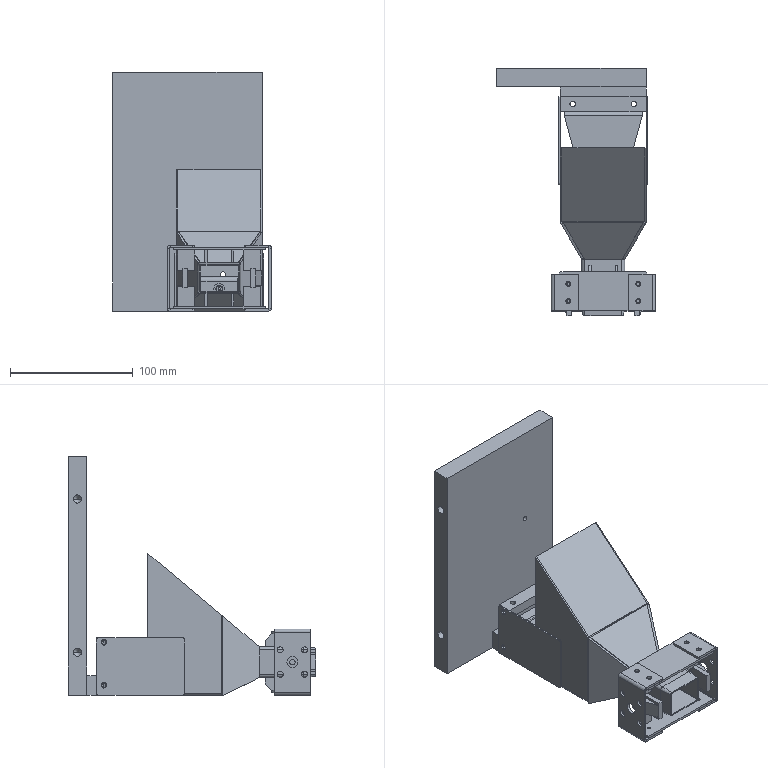Assembly | SolidWorks | mm | 12 component files | 29 solids | 449 faces | box 129.5 x 201.89 x 195.59 mm | volume 479848 mm3 | plane 263 | cylinder 162 | cone 18 | spline 4 | sphere 2 | commonest cylinder face diameters 4.5 x24 5 x24 4 x24 2.5 x16 3.3 x14 2 x14 1 x12 4.2 x8
Bill of materials:
InnerBagFunnel1 | 1 |  | Multi-body fabricated-style assembly: a rectangular hollow tube with rounded corners runs between two parallel flat plates, with small vertical rib plates between the plates. One end of the tube opens into a flared, pyramid-shaped (funnel-like) rectangular transition. The other end narrows slightly.
InnerBagFunnel2 | 1 |  | Bent thin-wall (sheet-like) part: a rectangular open channel or box section with one end cut at an angle, plus a flat tab extending sideways with two holes. A semicircular notch is cut into the edge of the bottom panel.
ClampingBlock | 2 |  | Solid prismatic block with a tapered lower profile, one round through-hole, a rectangular notch cut across the top edge, opposing notches on the sides, and a shallow rectangular recess or step on one face.
InnerBagClampingCylinderFixingPlate | 2 |  | U-shaped (C-channel) thin bracket with rounded bends. The web has one large central hole and four smaller holes in a rectangular pattern. Each of the two parallel flanges has two holes.
InnerBagLiftingAluminumBlockA | 1 |  | Rectangular solid bar with several cross-drilled holes: two holes through the top face near each end, two holes through a side face near each end, and one hole at the end face.
InnerBagLiftingAluminumBlockB | 1 |  | Rectangular solid bar with two through-holes in the top face near each end and one hole in an end face. No holes are visible on the long side face.
InnerBagLiftingCylinderFixingPlate | 1 |  | Flat rectangular plate with two small round holes, both near one long edge.
SiliconeShockAbsorberBlock | 1 |  | Plain rectangular solid bar with no visible holes or other features.
SmallRoundCylinderBracket | 1 |  | Bent thin bracket with a trapezoidal (tapered) top panel and two downturned legs with rounded bends. The legs have unequal lengths, and each has one round hole.
TeaSortingRod | 1 |  | Pin-like revolved part: a short cylindrical head with chamfered ends and a long, slender, coaxial cylindrical shaft ending in a rounded tip.
Mates:
1. coincident | InnerBagLiftingCylinderFixingPlate-1 face at (-22.646, -34.068, 148.933) dir (0, -1, 0) | assembly face at (71.854, 23.397, 163.933) dir (0, 0, -1)
2. concentric | InnerBagLiftingCylinderFixingPlate-1 face at (67.354, -34.068, 258.933) dir (0, -1, 0) r 2.1 | assembly face at (64.354, 133.397, 183.633) dir (0, 0, -1) r 2.6
3. concentric | InnerBagLiftingCylinderFixingPlate-1 face at (67.354, -34.068, 178.933) dir (0, -1, 0) r 2.1 | assembly face at (64.354, 53.397, 183.633) dir (0, 0, -1) r 2.6
4. coincident | assembly face at (33.354, -54.068, 187.933) dir (0, 0, 1) | InnerBagLiftingAluminumBlockB-1 face at (29.354, -54.068, 187.933) dir (0, 0, -1)
5. concentric | assembly face at (89.354, -48.068, 187.554) dir (0, 0, -1) r 1.621 | InnerBagLiftingAluminumBlockB-1 face at (89.354, -48.068, 187.933) dir (0, 0, 1) r 2.25
6. concentric | assembly face at (39.354, -48.068, 187.554) dir (0, 0, -1) r 1.621 | InnerBagLiftingAluminumBlockB-1 face at (39.354, -48.068, 187.933) dir (0, 0, 1) r 2.25
7. coincident | assembly face at (95.354, -54.068, 164.933) dir (0, 0, -1) | InnerBagLiftingAluminumBlockA-1 face at (29.354, -54.068, 164.933) dir (0, 0, 1)
8. concentric | InnerBagLiftingAluminumBlockA-1 face at (89.354, -48.068, 148.933) dir (0, 0, 1) r 2.25 | InnerBagLiftingAluminumBlockB-1 face at (89.354, -48.068, 187.933) dir (0, 0, 1) r 2.25
9. concentric | InnerBagLiftingAluminumBlockA-1 face at (39.354, -48.068, 148.933) dir (0, 0, 1) r 2.25 | InnerBagLiftingAluminumBlockB-1 face at (39.354, -48.068, 187.933) dir (0, 0, 1) r 2.25
10. coincident | InnerBagLiftingAluminumBlockA-1 face at (29.354, -54.068, 164.933) dir (0, -1, 0) | SmallRoundCylinderBracket-1 face at (96.354, -54.068, 176.933) dir (0, 1, 0)
11. concentric | InnerBagLiftingAluminumBlockA-1 face at (44.354, -42.068, 156.933) dir (0, 1, 0) r 1.65 | SmallRoundCylinderBracket-1 face at (44.354, -64.068, 156.933) dir (0, 1, 0) r 2.25
12. concentric | InnerBagLiftingAluminumBlockA-1 face at (84.354, -42.068, 156.933) dir (0, 1, 0) r 1.65 | SmallRoundCylinderBracket-1 face at (84.354, -64.068, 156.933) dir (0, 1, 0) r 2.25
13. coincident | InnerBagLiftingAluminumBlockA-1 face at (99.354, -54.068, 164.933) dir (1, 0, 0) | BAssemblyInnerBagFunnel-1/InnerBagFunnel2-1 face at (99.354, -112.068, 150.933) dir (-1, 0, 0)
14. concentric | InnerBagLiftingAluminumBlockA-1 face at (99.354, -48.068, 156.933) dir (1, 0, 0) r 1.65 | BAssemblyInnerBagFunnel-1/InnerBagFunnel2-1 face at (100.554, -48.068, 156.933) dir (-1, 0, 0) r 2.25
15. concentric | InnerBagLiftingAluminumBlockB-1 face at (99.354, -48.068, 191.933) dir (1, 0, 0) r 1.65 | BAssemblyInnerBagFunnel-1/InnerBagFunnel2-1 face at (100.554, -48.068, 191.933) dir (-1, 0, 0) r 2.25
16. concentric | BAssemblyInnerBagFunnel-1/InnerBagFunnel1-1 face at (92.854, -194.962, 150.844) dir (0, 0, -1) r 1.25 | InnerBagClampingCylinderFixingPlate-1 face at (92.854, -194.962, 148.844) dir (0, 0, 1) r 2
17. concentric | BAssemblyInnerBagFunnel-1/InnerBagFunnel1-1 face at (92.854, -208.962, 150.844) dir (0, 0, -1) r 1.25 | InnerBagClampingCylinderFixingPlate-1 face at (92.854, -208.962, 148.844) dir (0, 0, 1) r 2
18. coincident | BAssemblyInnerBagFunnel-1/InnerBagFunnel1-1 face at (64.354, -197.962, 150.844) dir (0, 0, -1) | InnerBagClampingCylinderFixingPlate-1 face at (104.854, -216.962, 150.844) dir (0, 0, 1)
19. parallel | BAssemblyInnerBagFunnel-1/InnerBagFunnel1-1 face at (98.354, -200.962, 169.344) dir (0, 1, 0) | ClampingBlock-1 face at (90.05, -193.962, 183.844) dir (0, 1, 0)
20. coincident | InnerBagLiftingAluminumBlockA-1 face at (29.354, -42.068, 164.933) dir (0, 1, 0) | SiliconeShockAbsorberBlock-1 face at (29.354, -42.068, 164.933) dir (0, -1, 0)
21. coincident | InnerBagLiftingAluminumBlockA-1 face at (29.354, -54.068, 148.933) dir (0, 0, -1) | SiliconeShockAbsorberBlock-1 face at (29.354, -42.068, 148.933) dir (0, 0, -1)
22. coincident | BAssemblyInnerBagFunnel-1/InnerBagFunnel2-1 face at (99.354, -112.068, 150.933) dir (-1, 0, 0) | SiliconeShockAbsorberBlock-1 face at (99.354, -42.068, 164.933) dir (1, 0, 0)
23. coincident | InnerBagLiftingCylinderFixingPlate-1 face at (-22.646, -34.068, 148.933) dir (0, -1, 0) | SiliconeShockAbsorberBlock-1 face at (29.354, -34.068, 164.933) dir (0, 1, 0)
24. coincident | InnerBagLiftingCylinderFixingPlate-1 face at (-22.646, -34.068, 148.933) dir (0, 0, -1) | SiliconeShockAbsorberBlock-1 face at (29.354, -42.068, 148.933) dir (0, 0, -1)
25. coincident | InnerBagLiftingCylinderFixingPlate-1 face at (99.354, -34.068, 148.933) dir (1, 0, 0) | SiliconeShockAbsorberBlock-1 face at (99.354, -42.068, 164.933) dir (1, 0, 0)
26. coincident | InnerBagFunnel1-1 edge at (49.518, 50.36, 41.807) dir (0, -1, 0) | InnerBagFunnel2-1 edge at (49.518, -15.624, 41.807) dir (0, 1, 0)
27. parallel | InnerBagFunnel1-1 face at (13.807, 2.676, 118.702) dir (0, 0, 1) | InnerBagFunnel2-1 face at (49.018, 50.976, 41.807) dir (0, 0, 1)
28. distance | InnerBagFunnel2-1 face at (50.718, 52.676, -18.193) dir (0, 1, 0) | InnerBagFunnel1-1 face at (13.807, 35.176, 118.702) dir (0, 1, 0)